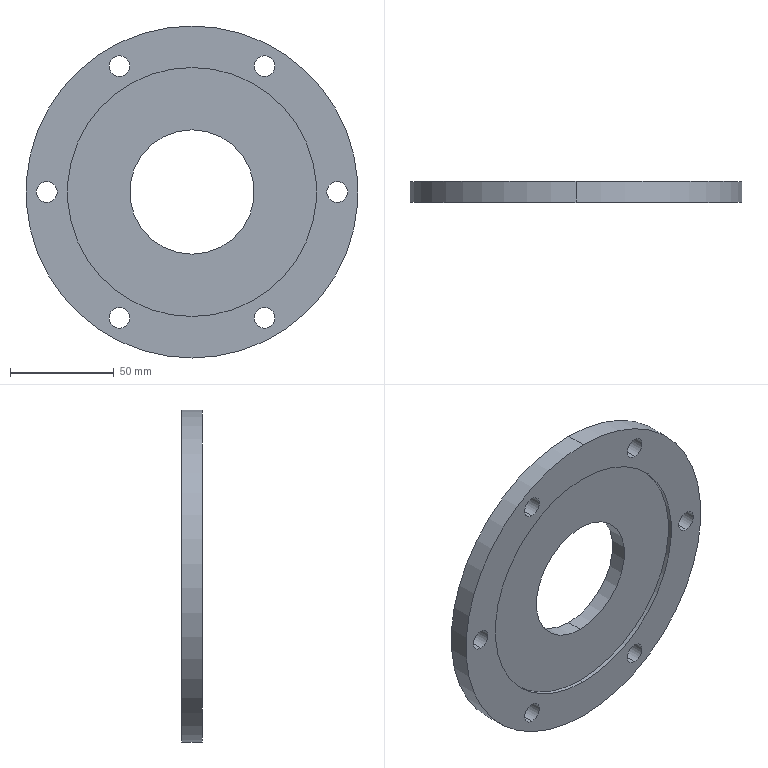Component | SolidWorks | GearboxEndCover-1 | 1 solid | 21 faces | box 160 x 10 x 160 mm | volume 151111 mm3 | cylinder 18 | plane 3 | commonest cylinder face diameters 10 x12 120 x2 160 x2 60 x2
build123d program:
from build123d import *

# Parameters (mm, degrees)
SKETCH1_3_R         = 80
SKETCH1_3_R_2       = 5
SKETCH1_3_R_3       = 30
BOSS_EXTRUDE1_DEPTH = 8
BOSS_EXTRUDE2_START = -2
SKETCH1_3_2_R       = 80
SKETCH1_3_2_R_2     = 60
SKETCH1_3_2_R_3     = 5
SKETCH1_3_2_R_4     = 30
BOSS_EXTRUDE2_DEPTH = 2


with BuildPart() as part:
    # Sketch1_3 → Boss-Extrude1 (new body)
    with BuildSketch(Plane(origin=(0, 0, 0), x_dir=(1, 0, 0), z_dir=(0, 1, 0))):
        with Locations(Location((0, 0, 0), (0, 0, 270))):
            Circle(SKETCH1_3_R)
        with Locations(Location((70, 0, 0), (0, 0, 270))):
            Circle(SKETCH1_3_R_2, mode=Mode.SUBTRACT)
        with Locations(Location((35, -60.622, 0), (0, 0, 270))):
            Circle(SKETCH1_3_R_2, mode=Mode.SUBTRACT)
        with Locations(Location((-35, -60.622, 0), (0, 0, 270))):
            Circle(SKETCH1_3_R_2, mode=Mode.SUBTRACT)
        with Locations(Location((-70, 0, 0), (0, 0, 270))):
            Circle(SKETCH1_3_R_2, mode=Mode.SUBTRACT)
        with Locations(Location((-35, 60.622, 0), (0, 0, 270))):
            Circle(SKETCH1_3_R_2, mode=Mode.SUBTRACT)
        with Locations(Location((35, 60.622, 0), (0, 0, 270))):
            Circle(SKETCH1_3_R_2, mode=Mode.SUBTRACT)
        with Locations(Location((0, 0, 0), (0, 0, 270))):
            Circle(SKETCH1_3_R_3, mode=Mode.SUBTRACT)
    extrude(amount=BOSS_EXTRUDE1_DEPTH)

    # Sketch1_3 2 → Boss-Extrude2 (add)
    # profile 1 of 2: a face of its own
    with BuildSketch(Plane(origin=(0, 0, 0), x_dir=(1, 0, 0), z_dir=(0, 1, 0)).offset(BOSS_EXTRUDE2_START)):
        with Locations(Location((0, 0, 0), (0, 0, 270))):
            Circle(SKETCH1_3_2_R)
        with Locations(Location((0, 0, 0), (0, 0, 270))):
            Circle(SKETCH1_3_2_R_2, mode=Mode.SUBTRACT)
        with Locations(Location((70, 0, 0), (0, 0, 270))):
            Circle(SKETCH1_3_2_R_3, mode=Mode.SUBTRACT)
        with Locations(Location((35, -60.622, 0), (0, 0, 270))):
            Circle(SKETCH1_3_2_R_3, mode=Mode.SUBTRACT)
        with Locations(Location((-35, -60.622, 0), (0, 0, 270))):
            Circle(SKETCH1_3_2_R_3, mode=Mode.SUBTRACT)
        with Locations(Location((-70, 0, 0), (0, 0, 270))):
            Circle(SKETCH1_3_2_R_3, mode=Mode.SUBTRACT)
        with Locations(Location((-35, 60.622, 0), (0, 0, 270))):
            Circle(SKETCH1_3_2_R_3, mode=Mode.SUBTRACT)
        with Locations(Location((35, 60.622, 0), (0, 0, 270))):
            Circle(SKETCH1_3_2_R_3, mode=Mode.SUBTRACT)
    # profile 2 of 2: a face of its own
    with BuildSketch(Plane(origin=(0, 0, 0), x_dir=(1, 0, 0), z_dir=(0, 1, 0)).offset(BOSS_EXTRUDE2_START)):
        with Locations(Location((0, 0, 0), (0, 0, 270))):
            Circle(SKETCH1_3_2_R_4)
    extrude(amount=BOSS_EXTRUDE2_DEPTH)


with BuildPart() as boss_extrude2_kept_piece:
    # of the separate pieces the step leaves, the one the design keeps (boss_extrude2_pieces_kept)
    add(part.part.solids().sort_by_distance((0, 8, 80))[0])


solid = boss_extrude2_kept_piece.part

# Placed as in the assembly
solid = solid.moved(Location((-40.429, -226.561, -5), (0, 0, 0)))
STEP:
#1=COLOUR_RGB('',0.7922,0.8196,0.9333);
#2=FILL_AREA_STYLE_COLOUR('',#1);
#3=FILL_AREA_STYLE('',(#2));
#4=SURFACE_STYLE_FILL_AREA(#3);
#5=SURFACE_SIDE_STYLE('',(#4));
#6=SURFACE_STYLE_USAGE(.BOTH.,#5);
#7=PRESENTATION_STYLE_ASSIGNMENT((#6));
#8=CARTESIAN_POINT('',(-1.592,-8.998,-2.559));
#9=VERTEX_POINT('',#8);
#10=CARTESIAN_POINT('',(-1.592,-8.998,2.165));
#11=VERTEX_POINT('',#10);
#12=CARTESIAN_POINT('',(-1.592,-8.998,-0.1969));
#13=DIRECTION('',(0.,1.,0.));
#14=DIRECTION('',(0.,0.,1.));
#15=AXIS2_PLACEMENT_3D('',#12,#13,#14);
#16=CIRCLE('',#15,2.362);
#17=EDGE_CURVE('',#9,#11,#16,.T.);
#18=ORIENTED_EDGE('',*,*,#17,.F.);
#19=CARTESIAN_POINT('',(-1.592,-8.92,-2.559));
#20=VERTEX_POINT('',#19);
#21=CARTESIAN_POINT('',(-1.592,-8.998,-2.559));
#22=DIRECTION('',(0.,1.,0.));
#23=VECTOR('',#22,39.37);
#24=LINE('',#21,#23);
#25=EDGE_CURVE('',#9,#20,#24,.T.);
#26=ORIENTED_EDGE('',*,*,#25,.T.);
#27=CARTESIAN_POINT('',(-1.592,-8.92,2.165));
#28=VERTEX_POINT('',#27);
#29=CARTESIAN_POINT('',(-1.592,-8.92,-0.1969));
#30=DIRECTION('',(0.,1.,0.));
#31=DIRECTION('',(0.,0.,1.));
#32=AXIS2_PLACEMENT_3D('',#29,#30,#31);
#33=CIRCLE('',#32,2.362);
#34=EDGE_CURVE('',#20,#28,#33,.T.);
#35=ORIENTED_EDGE('',*,*,#34,.T.);
#36=CARTESIAN_POINT('',(-1.592,-8.998,2.165));
#37=DIRECTION('',(0.,1.,0.));
#38=VECTOR('',#37,39.37);
#39=LINE('',#36,#38);
#40=EDGE_CURVE('',#11,#28,#39,.T.);
#41=ORIENTED_EDGE('',*,*,#40,.F.);
#42=EDGE_LOOP('',(#18,#26,#35,#41));
#43=FACE_OUTER_BOUND('',#42,.T.);
#44=CARTESIAN_POINT('',(-1.592,-8.998,-0.1969));
#45=DIRECTION('',(0.,1.,0.));
#46=DIRECTION('',(0.,0.,1.));
#47=AXIS2_PLACEMENT_3D('',#44,#45,#46);
#48=CYLINDRICAL_SURFACE('',#47,2.362);
#49=ADVANCED_FACE('',(#43),#48,.F.);
#50=CARTESIAN_POINT('',(-1.592,-8.605,2.953));
#51=VERTEX_POINT('',#50);
#52=CARTESIAN_POINT('',(-1.592,-8.605,-3.346));
#53=VERTEX_POINT('',#52);
#54=CARTESIAN_POINT('',(-1.592,-8.605,-0.1969));
#55=DIRECTION('',(0.,1.,0.));
#56=DIRECTION('',(0.,0.,1.));
#57=AXIS2_PLACEMENT_3D('',#54,#55,#56);
#58=CIRCLE('',#57,3.15);
#59=EDGE_CURVE('',#51,#53,#58,.T.);
#60=ORIENTED_EDGE('',*,*,#59,.F.);
#61=CARTESIAN_POINT('',(-1.592,-8.998,2.953));
#62=VERTEX_POINT('',#61);
#63=CARTESIAN_POINT('',(-1.592,-8.605,2.953));
#64=DIRECTION('',(0.,-1.,0.));
#65=VECTOR('',#64,39.37);
#66=LINE('',#63,#65);
#67=EDGE_CURVE('',#51,#62,#66,.T.);
#68=ORIENTED_EDGE('',*,*,#67,.T.);
#69=CARTESIAN_POINT('',(-1.592,-8.998,-3.346));
#70=VERTEX_POINT('',#69);
#71=CARTESIAN_POINT('',(-1.592,-8.998,-0.1969));
#72=DIRECTION('',(0.,1.,0.));
#73=DIRECTION('',(0.,0.,1.));
#74=AXIS2_PLACEMENT_3D('',#71,#72,#73);
#75=CIRCLE('',#74,3.15);
#76=EDGE_CURVE('',#62,#70,#75,.T.);
#77=ORIENTED_EDGE('',*,*,#76,.T.);
#78=CARTESIAN_POINT('',(-1.592,-8.605,-3.346));
#79=DIRECTION('',(0.,-1.,0.));
#80=VECTOR('',#79,39.37);
#81=LINE('',#78,#80);
#82=EDGE_CURVE('',#53,#70,#81,.T.);
#83=ORIENTED_EDGE('',*,*,#82,.F.);
#84=EDGE_LOOP('',(#60,#68,#77,#83));
#85=FACE_OUTER_BOUND('',#84,.T.);
#86=CARTESIAN_POINT('',(-1.592,-8.605,-0.1969));
#87=DIRECTION('',(0.,-1.,0.));
#88=DIRECTION('',(0.,0.,-1.));
#89=AXIS2_PLACEMENT_3D('',#86,#87,#88);
#90=CYLINDRICAL_SURFACE('',#89,3.15);
#91=ADVANCED_FACE('',(#85),#90,.T.);
#92=CARTESIAN_POINT('',(-1.592,-8.605,-1.378));
#93=VERTEX_POINT('',#92);
#94=CARTESIAN_POINT('',(-1.592,-8.605,0.9843));
#95=VERTEX_POINT('',#94);
#96=CARTESIAN_POINT('',(-1.592,-8.605,-0.1969));
#97=DIRECTION('',(0.,1.,0.));
#98=DIRECTION('',(0.,0.,1.));
#99=AXIS2_PLACEMENT_3D('',#96,#97,#98);
#100=CIRCLE('',#99,1.181);
#101=EDGE_CURVE('',#93,#95,#100,.T.);
#102=ORIENTED_EDGE('',*,*,#101,.T.);
#103=CARTESIAN_POINT('',(-1.592,-8.92,0.9843));
#104=VERTEX_POINT('',#103);
#105=CARTESIAN_POINT('',(-1.592,-8.605,0.9843));
#106=DIRECTION('',(0.,-1.,0.));
#107=VECTOR('',#106,39.37);
#108=LINE('',#105,#107);
#109=EDGE_CURVE('',#95,#104,#108,.T.);
#110=ORIENTED_EDGE('',*,*,#109,.T.);
#111=CARTESIAN_POINT('',(-1.592,-8.92,-1.378));
#112=VERTEX_POINT('',#111);
#113=CARTESIAN_POINT('',(-1.592,-8.92,-0.1969));
#114=DIRECTION('',(0.,1.,0.));
#115=DIRECTION('',(0.,0.,1.));
#116=AXIS2_PLACEMENT_3D('',#113,#114,#115);
#117=CIRCLE('',#116,1.181);
#118=EDGE_CURVE('',#112,#104,#117,.T.);
#119=ORIENTED_EDGE('',*,*,#118,.F.);
#120=CARTESIAN_POINT('',(-1.592,-8.605,-1.378));
#121=DIRECTION('',(0.,-1.,0.));
#122=VECTOR('',#121,39.37);
#123=LINE('',#120,#122);
#124=EDGE_CURVE('',#93,#112,#123,.T.);
#125=ORIENTED_EDGE('',*,*,#124,.F.);
#126=EDGE_LOOP('',(#102,#110,#119,#125));
#127=FACE_OUTER_BOUND('',#126,.T.);
#128=CARTESIAN_POINT('',(-1.592,-8.605,-0.1969));
#129=DIRECTION('',(0.,-1.,0.));
#130=DIRECTION('',(0.,0.,-1.));
#131=AXIS2_PLACEMENT_3D('',#128,#129,#130);
#132=CYLINDRICAL_SURFACE('',#131,1.181);
#133=ADVANCED_FACE('',(#127),#132,.F.);
#134=CARTESIAN_POINT('',(1.164,-8.605,-0.3937));
#135=VERTEX_POINT('',#134);
#136=CARTESIAN_POINT('',(1.164,-8.605,-0.));
#137=VERTEX_POINT('',#136);
#138=CARTESIAN_POINT('',(1.164,-8.605,-0.1969));
#139=DIRECTION('',(0.,1.,0.));
#140=DIRECTION('',(0.,0.,1.));
#141=AXIS2_PLACEMENT_3D('',#138,#139,#140);
#142=CIRCLE('',#141,0.1969);
#143=EDGE_CURVE('',#135,#137,#142,.T.);
#144=ORIENTED_EDGE('',*,*,#143,.T.);
#145=CARTESIAN_POINT('',(1.164,-8.998,-0.));
#146=VERTEX_POINT('',#145);
#147=CARTESIAN_POINT('',(1.164,-8.605,-0.));
#148=DIRECTION('',(0.,-1.,0.));
#149=VECTOR('',#148,39.37);
#150=LINE('',#147,#149);
#151=EDGE_CURVE('',#137,#146,#150,.T.);
#152=ORIENTED_EDGE('',*,*,#151,.T.);
#153=CARTESIAN_POINT('',(1.164,-8.998,-0.3937));
#154=VERTEX_POINT('',#153);
#155=CARTESIAN_POINT('',(1.164,-8.998,-0.1969));
#156=DIRECTION('',(0.,1.,0.));
#157=DIRECTION('',(0.,0.,1.));
#158=AXIS2_PLACEMENT_3D('',#155,#156,#157);
#159=CIRCLE('',#158,0.1969);
#160=EDGE_CURVE('',#154,#146,#159,.T.);
#161=ORIENTED_EDGE('',*,*,#160,.F.);
#162=CARTESIAN_POINT('',(1.164,-8.605,-0.3937));
#163=DIRECTION('',(0.,-1.,0.));
#164=VECTOR('',#163,39.37);
#165=LINE('',#162,#164);
#166=EDGE_CURVE('',#135,#154,#165,.T.);
#167=ORIENTED_EDGE('',*,*,#166,.F.);
#168=EDGE_LOOP('',(#144,#152,#161,#167));
#169=FACE_OUTER_BOUND('',#168,.T.);
#170=CARTESIAN_POINT('',(1.164,-8.605,-0.1969));
#171=DIRECTION('',(0.,-1.,0.));
#172=DIRECTION('',(0.,0.,-1.));
#173=AXIS2_PLACEMENT_3D('',#170,#171,#172);
#174=CYLINDRICAL_SURFACE('',#173,0.1969);
#175=ADVANCED_FACE('',(#169),#174,.F.);
#176=CARTESIAN_POINT('',(-0.2137,-8.605,-2.78));
#177=VERTEX_POINT('',#176);
#178=CARTESIAN_POINT('',(-0.2137,-8.605,-2.387));
#179=VERTEX_POINT('',#178);
#180=CARTESIAN_POINT('',(-0.2137,-8.605,-2.584));
#181=DIRECTION('',(0.,1.,0.));
#182=DIRECTION('',(0.,0.,1.));
#183=AXIS2_PLACEMENT_3D('',#180,#181,#182);
#184=CIRCLE('',#183,0.1969);
#185=EDGE_CURVE('',#177,#179,#184,.T.);
#186=ORIENTED_EDGE('',*,*,#185,.T.);
#187=CARTESIAN_POINT('',(-0.2137,-8.998,-2.387));
#188=VERTEX_POINT('',#187);
#189=CARTESIAN_POINT('',(-0.2137,-8.605,-2.387));
#190=DIRECTION('',(0.,-1.,0.));
#191=VECTOR('',#190,39.37);
#192=LINE('',#189,#191);
#193=EDGE_CURVE('',#179,#188,#192,.T.);
#194=ORIENTED_EDGE('',*,*,#193,.T.);
#195=CARTESIAN_POINT('',(-0.2137,-8.998,-2.78));
#196=VERTEX_POINT('',#195);
#197=CARTESIAN_POINT('',(-0.2137,-8.998,-2.584));
#198=DIRECTION('',(0.,1.,0.));
#199=DIRECTION('',(0.,0.,1.));
#200=AXIS2_PLACEMENT_3D('',#197,#198,#199);
#201=CIRCLE('',#200,0.1969);
#202=EDGE_CURVE('',#196,#188,#201,.T.);
#203=ORIENTED_EDGE('',*,*,#202,.F.);
#204=CARTESIAN_POINT('',(-0.2137,-8.605,-2.78));
#205=DIRECTION('',(0.,-1.,0.));
#206=VECTOR('',#205,39.37);
#207=LINE('',#204,#206);
#208=EDGE_CURVE('',#177,#196,#207,.T.);
#209=ORIENTED_EDGE('',*,*,#208,.F.);
#210=EDGE_LOOP('',(#186,#194,#203,#209));
#211=FACE_OUTER_BOUND('',#210,.T.);
#212=CARTESIAN_POINT('',(-0.2137,-8.605,-2.584));
#213=DIRECTION('',(0.,-1.,0.));
#214=DIRECTION('',(0.,0.,-1.));
#215=AXIS2_PLACEMENT_3D('',#212,#213,#214);
#216=CYLINDRICAL_SURFACE('',#215,0.1969);
#217=ADVANCED_FACE('',(#211),#216,.F.);
#218=CARTESIAN_POINT('',(-2.97,-8.605,-2.78));
#219=VERTEX_POINT('',#218);
#220=CARTESIAN_POINT('',(-2.97,-8.605,-2.387));
#221=VERTEX_POINT('',#220);
#222=CARTESIAN_POINT('',(-2.97,-8.605,-2.584));
#223=DIRECTION('',(0.,1.,0.));
#224=DIRECTION('',(0.,0.,1.));
#225=AXIS2_PLACEMENT_3D('',#222,#223,#224);
#226=CIRCLE('',#225,0.1969);
#227=EDGE_CURVE('',#219,#221,#226,.T.);
#228=ORIENTED_EDGE('',*,*,#227,.T.);
#229=CARTESIAN_POINT('',(-2.97,-8.998,-2.387));
#230=VERTEX_POINT('',#229);
#231=CARTESIAN_POINT('',(-2.97,-8.605,-2.387));
#232=DIRECTION('',(0.,-1.,0.));
#233=VECTOR('',#232,39.37);
#234=LINE('',#231,#233);
#235=EDGE_CURVE('',#221,#230,#234,.T.);
#236=ORIENTED_EDGE('',*,*,#235,.T.);
#237=CARTESIAN_POINT('',(-2.97,-8.998,-2.78));
#238=VERTEX_POINT('',#237);
#239=CARTESIAN_POINT('',(-2.97,-8.998,-2.584));
#240=DIRECTION('',(0.,1.,0.));
#241=DIRECTION('',(0.,0.,1.));
#242=AXIS2_PLACEMENT_3D('',#239,#240,#241);
#243=CIRCLE('',#242,0.1969);
#244=EDGE_CURVE('',#238,#230,#243,.T.);
#245=ORIENTED_EDGE('',*,*,#244,.F.);
#246=CARTESIAN_POINT('',(-2.97,-8.605,-2.78));
#247=DIRECTION('',(0.,-1.,0.));
#248=VECTOR('',#247,39.37);
#249=LINE('',#246,#248);
#250=EDGE_CURVE('',#219,#238,#249,.T.);
#251=ORIENTED_EDGE('',*,*,#250,.F.);
#252=EDGE_LOOP('',(#228,#236,#245,#251));
#253=FACE_OUTER_BOUND('',#252,.T.);
#254=CARTESIAN_POINT('',(-2.97,-8.605,-2.584));
#255=DIRECTION('',(0.,-1.,0.));
#256=DIRECTION('',(0.,0.,-1.));
#257=AXIS2_PLACEMENT_3D('',#254,#255,#256);
#258=CYLINDRICAL_SURFACE('',#257,0.1969);
#259=ADVANCED_FACE('',(#253),#258,.F.);
#260=CARTESIAN_POINT('',(-4.348,-8.605,-0.3937));
#261=VERTEX_POINT('',#260);
#262=CARTESIAN_POINT('',(-4.348,-8.605,-0.));
#263=VERTEX_POINT('',#262);
#264=CARTESIAN_POINT('',(-4.348,-8.605,-0.1969));
#265=DIRECTION('',(0.,1.,0.));
#266=DIRECTION('',(0.,0.,1.));
#267=AXIS2_PLACEMENT_3D('',#264,#265,#266);
#268=CIRCLE('',#267,0.1969);
#269=EDGE_CURVE('',#261,#263,#268,.T.);
#270=ORIENTED_EDGE('',*,*,#269,.T.);
#271=CARTESIAN_POINT('',(-4.348,-8.998,-0.));
#272=VERTEX_POINT('',#271);
#273=CARTESIAN_POINT('',(-4.348,-8.605,-0.));
#274=DIRECTION('',(0.,-1.,0.));
#275=VECTOR('',#274,39.37);
#276=LINE('',#273,#275);
#277=EDGE_CURVE('',#263,#272,#276,.T.);
#278=ORIENTED_EDGE('',*,*,#277,.T.);
#279=CARTESIAN_POINT('',(-4.348,-8.998,-0.3937));
#280=VERTEX_POINT('',#279);
#281=CARTESIAN_POINT('',(-4.348,-8.998,-0.1969));
#282=DIRECTION('',(0.,1.,0.));
#283=DIRECTION('',(0.,0.,1.));
#284=AXIS2_PLACEMENT_3D('',#281,#282,#283);
#285=CIRCLE('',#284,0.1969);
#286=EDGE_CURVE('',#280,#272,#285,.T.);
#287=ORIENTED_EDGE('',*,*,#286,.F.);
#288=CARTESIAN_POINT('',(-4.348,-8.605,-0.3937));
#289=DIRECTION('',(0.,-1.,0.));
#290=VECTOR('',#289,39.37);
#291=LINE('',#288,#290);
#292=EDGE_CURVE('',#261,#280,#291,.T.);
#293=ORIENTED_EDGE('',*,*,#292,.F.);
#294=EDGE_LOOP('',(#270,#278,#287,#293));
#295=FACE_OUTER_BOUND('',#294,.T.);
#296=CARTESIAN_POINT('',(-4.348,-8.605,-0.1969));
#297=DIRECTION('',(0.,-1.,0.));
#298=DIRECTION('',(0.,0.,-1.));
#299=AXIS2_PLACEMENT_3D('',#296,#297,#298);
#300=CYLINDRICAL_SURFACE('',#299,0.1969);
#301=ADVANCED_FACE('',(#295),#300,.F.);
#302=CARTESIAN_POINT('',(-2.97,-8.605,1.993));
#303=VERTEX_POINT('',#302);
#304=CARTESIAN_POINT('',(-2.97,-8.605,2.387));
#305=VERTEX_POINT('',#304);
#306=CARTESIAN_POINT('',(-2.97,-8.605,2.19));
#307=DIRECTION('',(0.,1.,0.));
#308=DIRECTION('',(0.,0.,1.));
#309=AXIS2_PLACEMENT_3D('',#306,#307,#308);
#310=CIRCLE('',#309,0.1969);
#311=EDGE_CURVE('',#303,#305,#310,.T.);
#312=ORIENTED_EDGE('',*,*,#311,.T.);
#313=CARTESIAN_POINT('',(-2.97,-8.998,2.387));
#314=VERTEX_POINT('',#313);
#315=CARTESIAN_POINT('',(-2.97,-8.605,2.387));
#316=DIRECTION('',(0.,-1.,0.));
#317=VECTOR('',#316,39.37);
#318=LINE('',#315,#317);
#319=EDGE_CURVE('',#305,#314,#318,.T.);
#320=ORIENTED_EDGE('',*,*,#319,.T.);
#321=CARTESIAN_POINT('',(-2.97,-8.998,1.993));
#322=VERTEX_POINT('',#321);
#323=CARTESIAN_POINT('',(-2.97,-8.998,2.19));
#324=DIRECTION('',(0.,1.,0.));
#325=DIRECTION('',(0.,0.,1.));
#326=AXIS2_PLACEMENT_3D('',#323,#324,#325);
#327=CIRCLE('',#326,0.1969);
#328=EDGE_CURVE('',#322,#314,#327,.T.);
#329=ORIENTED_EDGE('',*,*,#328,.F.);
#330=CARTESIAN_POINT('',(-2.97,-8.605,1.993));
#331=DIRECTION('',(0.,-1.,0.));
#332=VECTOR('',#331,39.37);
#333=LINE('',#330,#332);
#334=EDGE_CURVE('',#303,#322,#333,.T.);
#335=ORIENTED_EDGE('',*,*,#334,.F.);
#336=EDGE_LOOP('',(#312,#320,#329,#335));
#337=FACE_OUTER_BOUND('',#336,.T.);
#338=CARTESIAN_POINT('',(-2.97,-8.605,2.19));
#339=DIRECTION('',(0.,-1.,0.));
#340=DIRECTION('',(0.,0.,-1.));
#341=AXIS2_PLACEMENT_3D('',#338,#339,#340);
#342=CYLINDRICAL_SURFACE('',#341,0.1969);
#343=ADVANCED_FACE('',(#337),#342,.F.);
#344=CARTESIAN_POINT('',(-0.2137,-8.605,1.993));
#345=VERTEX_POINT('',#344);
#346=CARTESIAN_POINT('',(-0.2137,-8.605,2.387));
#347=VERTEX_POINT('',#346);
#348=CARTESIAN_POINT('',(-0.2137,-8.605,2.19));
#349=DIRECTION('',(0.,1.,0.));
#350=DIRECTION('',(0.,0.,1.));
#351=AXIS2_PLACEMENT_3D('',#348,#349,#350);
#352=CIRCLE('',#351,0.1969);
#353=EDGE_CURVE('',#345,#347,#352,.T.);
#354=ORIENTED_EDGE('',*,*,#353,.T.);
#355=CARTESIAN_POINT('',(-0.2137,-8.998,2.387));
#356=VERTEX_POINT('',#355);
#357=CARTESIAN_POINT('',(-0.2137,-8.605,2.387));
#358=DIRECTION('',(0.,-1.,0.));
#359=VECTOR('',#358,39.37);
#360=LINE('',#357,#359);
#361=EDGE_CURVE('',#347,#356,#360,.T.);
#362=ORIENTED_EDGE('',*,*,#361,.T.);
#363=CARTESIAN_POINT('',(-0.2137,-8.998,1.993));
#364=VERTEX_POINT('',#363);
#365=CARTESIAN_POINT('',(-0.2137,-8.998,2.19));
#366=DIRECTION('',(0.,1.,0.));
#367=DIRECTION('',(0.,0.,1.));
#368=AXIS2_PLACEMENT_3D('',#365,#366,#367);
#369=CIRCLE('',#368,0.1969);
#370=EDGE_CURVE('',#364,#356,#369,.T.);
#371=ORIENTED_EDGE('',*,*,#370,.F.);
#372=CARTESIAN_POINT('',(-0.2137,-8.605,1.993));
#373=DIRECTION('',(0.,-1.,0.));
#374=VECTOR('',#373,39.37);
#375=LINE('',#372,#374);
#376=EDGE_CURVE('',#345,#364,#375,.T.);
#377=ORIENTED_EDGE('',*,*,#376,.F.);
#378=EDGE_LOOP('',(#354,#362,#371,#377));
#379=FACE_OUTER_BOUND('',#378,.T.);
#380=CARTESIAN_POINT('',(-0.2137,-8.605,2.19));
#381=DIRECTION('',(0.,-1.,0.));
#382=DIRECTION('',(0.,0.,-1.));
#383=AXIS2_PLACEMENT_3D('',#380,#381,#382);
#384=CYLINDRICAL_SURFACE('',#383,0.1969);
#385=ADVANCED_FACE('',(#379),#384,.F.);
#386=ORIENTED_EDGE('',*,*,#118,.T.);
#387=CARTESIAN_POINT('',(-1.592,-8.92,-0.1969));
#388=DIRECTION('',(0.,1.,0.));
#389=DIRECTION('',(0.,0.,1.));
#390=AXIS2_PLACEMENT_3D('',#387,#388,#389);
#391=CIRCLE('',#390,1.181);
#392=EDGE_CURVE('',#104,#112,#391,.T.);
#393=ORIENTED_EDGE('',*,*,#392,.T.);
#394=EDGE_LOOP('',(#386,#393));
#395=FACE_BOUND('',#394,.T.);
#396=CARTESIAN_POINT('',(-1.592,-8.92,-0.1969));
#397=DIRECTION('',(0.,1.,0.));
#398=DIRECTION('',(0.,0.,1.));
#399=AXIS2_PLACEMENT_3D('',#396,#397,#398);
#400=CIRCLE('',#399,2.362);
#401=EDGE_CURVE('',#28,#20,#400,.T.);
#402=ORIENTED_EDGE('',*,*,#401,.F.);
#403=ORIENTED_EDGE('',*,*,#34,.F.);
#404=EDGE_LOOP('',(#402,#403));
#405=FACE_OUTER_BOUND('',#404,.T.);
#406=CARTESIAN_POINT('',(-8.526,-8.92,-0.1969));
#407=DIRECTION('',(0.,1.,0.));
#408=DIRECTION('',(0.,0.,1.));
#409=AXIS2_PLACEMENT_3D('',#406,#407,#408);
#410=PLANE('',#409);
#411=ADVANCED_FACE('',(#395,#405),#410,.F.);
#412=ORIENTED_EDGE('',*,*,#361,.F.);
#413=CARTESIAN_POINT('',(-0.2137,-8.605,2.19));
#414=DIRECTION('',(0.,1.,0.));
#415=DIRECTION('',(0.,0.,1.));
#416=AXIS2_PLACEMENT_3D('',#413,#414,#415);
#417=CIRCLE('',#416,0.1969);
#418=EDGE_CURVE('',#347,#345,#417,.T.);
#419=ORIENTED_EDGE('',*,*,#418,.T.);
#420=ORIENTED_EDGE('',*,*,#376,.T.);
#421=CARTESIAN_POINT('',(-0.2137,-8.998,2.19));
#422=DIRECTION('',(0.,1.,0.));
#423=DIRECTION('',(0.,0.,1.));
#424=AXIS2_PLACEMENT_3D('',#421,#422,#423);
#425=CIRCLE('',#424,0.1969);
#426=EDGE_CURVE('',#356,#364,#425,.T.);
#427=ORIENTED_EDGE('',*,*,#426,.F.);
#428=EDGE_LOOP('',(#412,#419,#420,#427));
#429=FACE_OUTER_BOUND('',#428,.T.);
#430=CARTESIAN_POINT('',(-0.2137,-8.605,2.19));
#431=DIRECTION('',(0.,-1.,0.));
#432=DIRECTION('',(0.,0.,-1.));
#433=AXIS2_PLACEMENT_3D('',#430,#431,#432);
#434=CYLINDRICAL_SURFACE('',#433,0.1969);
#435=ADVANCED_FACE('',(#429),#434,.F.);
#436=ORIENTED_EDGE('',*,*,#319,.F.);
#437=CARTESIAN_POINT('',(-2.97,-8.605,2.19));
#438=DIRECTION('',(0.,1.,0.));
#439=DIRECTION('',(0.,0.,1.));
#440=AXIS2_PLACEMENT_3D('',#437,#438,#439);
#441=CIRCLE('',#440,0.1969);
#442=EDGE_CURVE('',#305,#303,#441,.T.);
#443=ORIENTED_EDGE('',*,*,#442,.T.);
#444=ORIENTED_EDGE('',*,*,#334,.T.);
#445=CARTESIAN_POINT('',(-2.97,-8.998,2.19));
#446=DIRECTION('',(0.,1.,0.));
#447=DIRECTION('',(0.,0.,1.));
#448=AXIS2_PLACEMENT_3D('',#445,#446,#447);
#449=CIRCLE('',#448,0.1969);
#450=EDGE_CURVE('',#314,#322,#449,.T.);
#451=ORIENTED_EDGE('',*,*,#450,.F.);
#452=EDGE_LOOP('',(#436,#443,#444,#451));
#453=FACE_OUTER_BOUND('',#452,.T.);
#454=CARTESIAN_POINT('',(-2.97,-8.605,2.19));
#455=DIRECTION('',(0.,-1.,0.));
#456=DIRECTION('',(0.,0.,-1.));
#457=AXIS2_PLACEMENT_3D('',#454,#455,#456);
#458=CYLINDRICAL_SURFACE('',#457,0.1969);
#459=ADVANCED_FACE('',(#453),#458,.F.);
#460=ORIENTED_EDGE('',*,*,#277,.F.);
#461=CARTESIAN_POINT('',(-4.348,-8.605,-0.1969));
#462=DIRECTION('',(0.,1.,0.));
#463=DIRECTION('',(0.,0.,1.));
#464=AXIS2_PLACEMENT_3D('',#461,#462,#463);
#465=CIRCLE('',#464,0.1969);
#466=EDGE_CURVE('',#263,#261,#465,.T.);
#467=ORIENTED_EDGE('',*,*,#466,.T.);
#468=ORIENTED_EDGE('',*,*,#292,.T.);
#469=CARTESIAN_POINT('',(-4.348,-8.998,-0.1969));
#470=DIRECTION('',(0.,1.,0.));
#471=DIRECTION('',(0.,0.,1.));
#472=AXIS2_PLACEMENT_3D('',#469,#470,#471);
#473=CIRCLE('',#472,0.1969);
#474=EDGE_CURVE('',#272,#280,#473,.T.);
#475=ORIENTED_EDGE('',*,*,#474,.F.);
#476=EDGE_LOOP('',(#460,#467,#468,#475));
#477=FACE_OUTER_BOUND('',#476,.T.);
#478=CARTESIAN_POINT('',(-4.348,-8.605,-0.1969));
#479=DIRECTION('',(0.,-1.,0.));
#480=DIRECTION('',(0.,0.,-1.));
#481=AXIS2_PLACEMENT_3D('',#478,#479,#480);
#482=CYLINDRICAL_SURFACE('',#481,0.1969);
#483=ADVANCED_FACE('',(#477),#482,.F.);
#484=ORIENTED_EDGE('',*,*,#235,.F.);
#485=CARTESIAN_POINT('',(-2.97,-8.605,-2.584));
#486=DIRECTION('',(0.,1.,0.));
#487=DIRECTION('',(0.,0.,1.));
#488=AXIS2_PLACEMENT_3D('',#485,#486,#487);
#489=CIRCLE('',#488,0.1969);
#490=EDGE_CURVE('',#221,#219,#489,.T.);
#491=ORIENTED_EDGE('',*,*,#490,.T.);
#492=ORIENTED_EDGE('',*,*,#250,.T.);
#493=CARTESIAN_POINT('',(-2.97,-8.998,-2.584));
#494=DIRECTION('',(0.,1.,0.));
#495=DIRECTION('',(0.,0.,1.));
#496=AXIS2_PLACEMENT_3D('',#493,#494,#495);
#497=CIRCLE('',#496,0.1969);
#498=EDGE_CURVE('',#230,#238,#497,.T.);
#499=ORIENTED_EDGE('',*,*,#498,.F.);
#500=EDGE_LOOP('',(#484,#491,#492,#499));
#501=FACE_OUTER_BOUND('',#500,.T.);
#502=CARTESIAN_POINT('',(-2.97,-8.605,-2.584));
#503=DIRECTION('',(0.,-1.,0.));
#504=DIRECTION('',(0.,0.,-1.));
#505=AXIS2_PLACEMENT_3D('',#502,#503,#504);
#506=CYLINDRICAL_SURFACE('',#505,0.1969);
#507=ADVANCED_FACE('',(#501),#506,.F.);
#508=ORIENTED_EDGE('',*,*,#193,.F.);
#509=CARTESIAN_POINT('',(-0.2137,-8.605,-2.584));
#510=DIRECTION('',(0.,1.,0.));
#511=DIRECTION('',(0.,0.,1.));
#512=AXIS2_PLACEMENT_3D('',#509,#510,#511);
#513=CIRCLE('',#512,0.1969);
#514=EDGE_CURVE('',#179,#177,#513,.T.);
#515=ORIENTED_EDGE('',*,*,#514,.T.);
#516=ORIENTED_EDGE('',*,*,#208,.T.);
#517=CARTESIAN_POINT('',(-0.2137,-8.998,-2.584));
#518=DIRECTION('',(0.,1.,0.));
#519=DIRECTION('',(0.,0.,1.));
#520=AXIS2_PLACEMENT_3D('',#517,#518,#519);
#521=CIRCLE('',#520,0.1969);
#522=EDGE_CURVE('',#188,#196,#521,.T.);
#523=ORIENTED_EDGE('',*,*,#522,.F.);
#524=EDGE_LOOP('',(#508,#515,#516,#523));
#525=FACE_OUTER_BOUND('',#524,.T.);
#526=CARTESIAN_POINT('',(-0.2137,-8.605,-2.584));
#527=DIRECTION('',(0.,-1.,0.));
#528=DIRECTION('',(0.,0.,-1.));
#529=AXIS2_PLACEMENT_3D('',#526,#527,#528);
#530=CYLINDRICAL_SURFACE('',#529,0.1969);
#531=ADVANCED_FACE('',(#525),#530,.F.);
#532=ORIENTED_EDGE('',*,*,#151,.F.);
#533=CARTESIAN_POINT('',(1.164,-8.605,-0.1969));
#534=DIRECTION('',(0.,1.,0.));
#535=DIRECTION('',(0.,0.,1.));
#536=AXIS2_PLACEMENT_3D('',#533,#534,#535);
#537=CIRCLE('',#536,0.1969);
#538=EDGE_CURVE('',#137,#135,#537,.T.);
#539=ORIENTED_EDGE('',*,*,#538,.T.);
#540=ORIENTED_EDGE('',*,*,#166,.T.);
#541=CARTESIAN_POINT('',(1.164,-8.998,-0.1969));
#542=DIRECTION('',(0.,1.,0.));
#543=DIRECTION('',(0.,0.,1.));
#544=AXIS2_PLACEMENT_3D('',#541,#542,#543);
#545=CIRCLE('',#544,0.1969);
#546=EDGE_CURVE('',#146,#154,#545,.T.);
#547=ORIENTED_EDGE('',*,*,#546,.F.);
#548=EDGE_LOOP('',(#532,#539,#540,#547));
#549=FACE_OUTER_BOUND('',#548,.T.);
#550=CARTESIAN_POINT('',(1.164,-8.605,-0.1969));
#551=DIRECTION('',(0.,-1.,0.));
#552=DIRECTION('',(0.,0.,-1.));
#553=AXIS2_PLACEMENT_3D('',#550,#551,#552);
#554=CYLINDRICAL_SURFACE('',#553,0.1969);
#555=ADVANCED_FACE('',(#549),#554,.F.);
#556=ORIENTED_EDGE('',*,*,#109,.F.);
#557=CARTESIAN_POINT('',(-1.592,-8.605,-0.1969));
#558=DIRECTION('',(0.,1.,0.));
#559=DIRECTION('',(0.,0.,1.));
#560=AXIS2_PLACEMENT_3D('',#557,#558,#559);
#561=CIRCLE('',#560,1.181);
#562=EDGE_CURVE('',#95,#93,#561,.T.);
#563=ORIENTED_EDGE('',*,*,#562,.T.);
#564=ORIENTED_EDGE('',*,*,#124,.T.);
#565=ORIENTED_EDGE('',*,*,#392,.F.);
#566=EDGE_LOOP('',(#556,#563,#564,#565));
#567=FACE_OUTER_BOUND('',#566,.T.);
#568=CARTESIAN_POINT('',(-1.592,-8.605,-0.1969));
#569=DIRECTION('',(0.,-1.,0.));
#570=DIRECTION('',(0.,0.,-1.));
#571=AXIS2_PLACEMENT_3D('',#568,#569,#570);
#572=CYLINDRICAL_SURFACE('',#571,1.181);
#573=ADVANCED_FACE('',(#567),#572,.F.);
#574=ORIENTED_EDGE('',*,*,#67,.F.);
#575=CARTESIAN_POINT('',(-1.592,-8.605,-0.1969));
#576=DIRECTION('',(0.,1.,0.));
#577=DIRECTION('',(0.,0.,1.));
#578=AXIS2_PLACEMENT_3D('',#575,#576,#577);
#579=CIRCLE('',#578,3.15);
#580=EDGE_CURVE('',#53,#51,#579,.T.);
#581=ORIENTED_EDGE('',*,*,#580,.F.);
#582=ORIENTED_EDGE('',*,*,#82,.T.);
#583=CARTESIAN_POINT('',(-1.592,-8.998,-0.1969));
#584=DIRECTION('',(0.,1.,0.));
#585=DIRECTION('',(0.,0.,1.));
#586=AXIS2_PLACEMENT_3D('',#583,#584,#585);
#587=CIRCLE('',#586,3.15);
#588=EDGE_CURVE('',#70,#62,#587,.T.);
#589=ORIENTED_EDGE('',*,*,#588,.T.);
#590=EDGE_LOOP('',(#574,#581,#582,#589));
#591=FACE_OUTER_BOUND('',#590,.T.);
#592=CARTESIAN_POINT('',(-1.592,-8.605,-0.1969));
#593=DIRECTION('',(0.,-1.,0.));
#594=DIRECTION('',(0.,0.,-1.));
#595=AXIS2_PLACEMENT_3D('',#592,#593,#594);
#596=CYLINDRICAL_SURFACE('',#595,3.15);
#597=ADVANCED_FACE('',(#591),#596,.T.);
#598=ORIENTED_EDGE('',*,*,#101,.F.);
#599=ORIENTED_EDGE('',*,*,#562,.F.);
#600=EDGE_LOOP('',(#598,#599));
#601=FACE_BOUND('',#600,.T.);
#602=ORIENTED_EDGE('',*,*,#143,.F.);
#603=ORIENTED_EDGE('',*,*,#538,.F.);
#604=EDGE_LOOP('',(#602,#603));
#605=FACE_BOUND('',#604,.T.);
#606=ORIENTED_EDGE('',*,*,#185,.F.);
#607=ORIENTED_EDGE('',*,*,#514,.F.);
#608=EDGE_LOOP('',(#606,#607));
#609=FACE_BOUND('',#608,.T.);
#610=ORIENTED_EDGE('',*,*,#227,.F.);
#611=ORIENTED_EDGE('',*,*,#490,.F.);
#612=EDGE_LOOP('',(#610,#611));
#613=FACE_BOUND('',#612,.T.);
#614=ORIENTED_EDGE('',*,*,#269,.F.);
#615=ORIENTED_EDGE('',*,*,#466,.F.);
#616=EDGE_LOOP('',(#614,#615));
#617=FACE_BOUND('',#616,.T.);
#618=ORIENTED_EDGE('',*,*,#311,.F.);
#619=ORIENTED_EDGE('',*,*,#442,.F.);
#620=EDGE_LOOP('',(#618,#619));
#621=FACE_BOUND('',#620,.T.);
#622=ORIENTED_EDGE('',*,*,#353,.F.);
#623=ORIENTED_EDGE('',*,*,#418,.F.);
#624=EDGE_LOOP('',(#622,#623));
#625=FACE_BOUND('',#624,.T.);
#626=ORIENTED_EDGE('',*,*,#580,.T.);
#627=ORIENTED_EDGE('',*,*,#59,.T.);
#628=EDGE_LOOP('',(#626,#627));
#629=FACE_OUTER_BOUND('',#628,.T.);
#630=CARTESIAN_POINT('',(-8.526,-8.605,-0.1969));
#631=DIRECTION('',(0.,1.,0.));
#632=DIRECTION('',(0.,0.,1.));
#633=AXIS2_PLACEMENT_3D('',#630,#631,#632);
#634=PLANE('',#633);
#635=ADVANCED_FACE('',(#601,#605,#609,#613,#617,#621,#625,#629),#634,.T.);
#636=ORIENTED_EDGE('',*,*,#25,.F.);
#637=CARTESIAN_POINT('',(-1.592,-8.998,-0.1969));
#638=DIRECTION('',(0.,1.,0.));
#639=DIRECTION('',(0.,0.,1.));
#640=AXIS2_PLACEMENT_3D('',#637,#638,#639);
#641=CIRCLE('',#640,2.362);
#642=EDGE_CURVE('',#11,#9,#641,.T.);
#643=ORIENTED_EDGE('',*,*,#642,.F.);
#644=ORIENTED_EDGE('',*,*,#40,.T.);
#645=ORIENTED_EDGE('',*,*,#401,.T.);
#646=EDGE_LOOP('',(#636,#643,#644,#645));
#647=FACE_OUTER_BOUND('',#646,.T.);
#648=CARTESIAN_POINT('',(-1.592,-8.998,-0.1969));
#649=DIRECTION('',(0.,1.,0.));
#650=DIRECTION('',(0.,0.,1.));
#651=AXIS2_PLACEMENT_3D('',#648,#649,#650);
#652=CYLINDRICAL_SURFACE('',#651,2.362);
#653=ADVANCED_FACE('',(#647),#652,.F.);
#654=ORIENTED_EDGE('',*,*,#160,.T.);
#655=ORIENTED_EDGE('',*,*,#546,.T.);
#656=EDGE_LOOP('',(#654,#655));
#657=FACE_BOUND('',#656,.T.);
#658=ORIENTED_EDGE('',*,*,#202,.T.);
#659=ORIENTED_EDGE('',*,*,#522,.T.);
#660=EDGE_LOOP('',(#658,#659));
#661=FACE_BOUND('',#660,.T.);
#662=ORIENTED_EDGE('',*,*,#244,.T.);
#663=ORIENTED_EDGE('',*,*,#498,.T.);
#664=EDGE_LOOP('',(#662,#663));
#665=FACE_BOUND('',#664,.T.);
#666=ORIENTED_EDGE('',*,*,#286,.T.);
#667=ORIENTED_EDGE('',*,*,#474,.T.);
#668=EDGE_LOOP('',(#666,#667));
#669=FACE_BOUND('',#668,.T.);
#670=ORIENTED_EDGE('',*,*,#328,.T.);
#671=ORIENTED_EDGE('',*,*,#450,.T.);
#672=EDGE_LOOP('',(#670,#671));
#673=FACE_BOUND('',#672,.T.);
#674=ORIENTED_EDGE('',*,*,#370,.T.);
#675=ORIENTED_EDGE('',*,*,#426,.T.);
#676=EDGE_LOOP('',(#674,#675));
#677=FACE_BOUND('',#676,.T.);
#678=ORIENTED_EDGE('',*,*,#642,.T.);
#679=ORIENTED_EDGE('',*,*,#17,.T.);
#680=EDGE_LOOP('',(#678,#679));
#681=FACE_BOUND('',#680,.T.);
#682=ORIENTED_EDGE('',*,*,#588,.F.);
#683=ORIENTED_EDGE('',*,*,#76,.F.);
#684=EDGE_LOOP('',(#682,#683));
#685=FACE_OUTER_BOUND('',#684,.T.);
#686=CARTESIAN_POINT('',(-8.526,-8.998,-0.1969));
#687=DIRECTION('',(0.,1.,0.));
#688=DIRECTION('',(0.,0.,1.));
#689=AXIS2_PLACEMENT_3D('',#686,#687,#688);
#690=PLANE('',#689);
#691=ADVANCED_FACE('',(#657,#661,#665,#669,#673,#677,#681,#685),#690,.F.);
#692=CLOSED_SHELL('',(#49,#91,#133,#175,#217,#259,#301,#343,#385,#411,#435,#459,#483,#507,#531,#555,#573,#597,#635,#653,#691));
#693=MANIFOLD_SOLID_BREP('',#692);
#694=STYLED_ITEM('',(#7),#693);
#695=PRESENTATION_LAYER_ASSIGNMENT('','',(#694));
#696=(LENGTH_UNIT()NAMED_UNIT(*)SI_UNIT($,.METRE.));
#697=LENGTH_MEASURE_WITH_UNIT(LENGTH_MEASURE(0.0254),#696);
#698=DIMENSIONAL_EXPONENTS(1.,0.,0.,0.,0.,0.,0.);
#699=(CONVERSION_BASED_UNIT('',#697)LENGTH_UNIT()NAMED_UNIT(#698));
#700=UNCERTAINTY_MEASURE_WITH_UNIT(LENGTH_MEASURE(0.00001),#699,'','');
#701=(NAMED_UNIT(*)PLANE_ANGLE_UNIT()SI_UNIT($,.RADIAN.));
#702=(NAMED_UNIT(*)SI_UNIT($,.STERADIAN.)SOLID_ANGLE_UNIT());
#703=(GEOMETRIC_REPRESENTATION_CONTEXT(3)GLOBAL_UNCERTAINTY_ASSIGNED_CONTEXT((#700))GLOBAL_UNIT_ASSIGNED_CONTEXT((#699,#701,#702))REPRESENTATION_CONTEXT('',''));
#704=MECHANICAL_DESIGN_GEOMETRIC_PRESENTATION_REPRESENTATION('',(#694),#703);
#705=CARTESIAN_POINT('',(0.,0.,0.));
#706=DIRECTION('',(0.,0.,1.));
#707=DIRECTION('',(1.,0.,0.));
#708=AXIS2_PLACEMENT_3D('',#705,#706,#707);
#709=(LENGTH_UNIT()NAMED_UNIT(*)SI_UNIT($,.METRE.));
#710=LENGTH_MEASURE_WITH_UNIT(LENGTH_MEASURE(0.0254),#709);
#711=DIMENSIONAL_EXPONENTS(1.,0.,0.,0.,0.,0.,0.);
#712=(CONVERSION_BASED_UNIT('',#710)LENGTH_UNIT()NAMED_UNIT(#711));
#713=UNCERTAINTY_MEASURE_WITH_UNIT(LENGTH_MEASURE(0.00001),#712,'','');
#714=(NAMED_UNIT(*)PLANE_ANGLE_UNIT()SI_UNIT($,.RADIAN.));
#715=(NAMED_UNIT(*)SI_UNIT($,.STERADIAN.)SOLID_ANGLE_UNIT());
#716=(GEOMETRIC_REPRESENTATION_CONTEXT(3)GLOBAL_UNCERTAINTY_ASSIGNED_CONTEXT((#713))GLOBAL_UNIT_ASSIGNED_CONTEXT((#712,#714,#715))REPRESENTATION_CONTEXT('',''));
#717=ADVANCED_BREP_SHAPE_REPRESENTATION('',(#693,#708),#716);